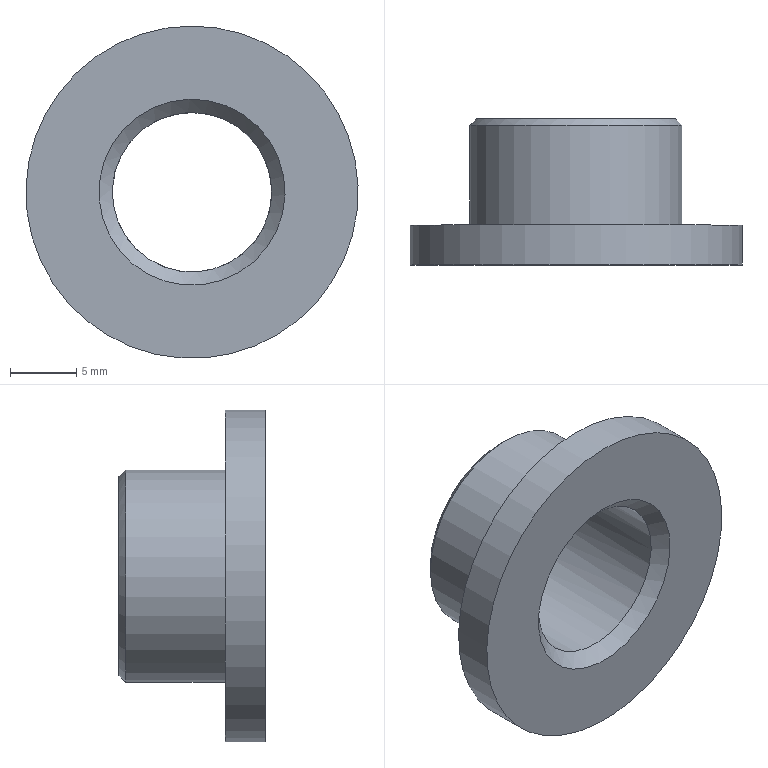Component | NX | CLHKJG_14_SHAFT_SLEEVE | 1 solid | 8 faces | box 25 x 11 x 25 mm | volume 1811 mm3 | plane 3 | cylinder 3 | cone 2 | commonest cylinder face diameters 25 x1 16 x1 12 x1
STEP:
#1=CARTESIAN_POINT('',(0.,0.,0.));
#2=DIRECTION('',(0.,0.,1.));
#3=DIRECTION('',(1.,0.,0.));
#4=AXIS2_PLACEMENT_3D('',#1,#2,#3);
#5=CARTESIAN_POINT('',(-367.568,64.665,-91.876));
#6=VERTEX_POINT('',#5);
#7=CARTESIAN_POINT('',(-360.87,64.665,-87.5));
#8=DIRECTION('',(0.,1.,0.));
#9=DIRECTION('',(-0.8372,0.,-0.5469));
#10=AXIS2_PLACEMENT_3D('',#7,#8,#9);
#11=CIRCLE('',#10,8.);
#12=CARTESIAN_POINT('',(-360.87,64.665,-87.5));
#13=DIRECTION('',(0.,1.,0.));
#14=DIRECTION('',(-0.8372,0.,-0.5469));
#15=AXIS2_PLACEMENT_3D('',#12,#13,#14);
#16=PLANE('',#15);
#17=CARTESIAN_POINT('',(0.,0.));
#18=DIRECTION('',(1.,0.));
#19=AXIS2_PLACEMENT_2D('',#17,#18);
#20=CIRCLE('',#19,8.);
#21=(GEOMETRIC_REPRESENTATION_CONTEXT(2)PARAMETRIC_REPRESENTATION_CONTEXT()REPRESENTATION_CONTEXT('',''));
#22=DEFINITIONAL_REPRESENTATION('',(#20),#21);
#23=PCURVE('',#16,#22);
#24=CARTESIAN_POINT('',(-360.87,64.665,-87.5));
#25=DIRECTION('',(0.,1.,0.));
#26=DIRECTION('',(-0.8372,0.,-0.5469));
#27=AXIS2_PLACEMENT_3D('',#24,#25,#26);
#28=CYLINDRICAL_SURFACE('',#27,8.);
#29=CARTESIAN_POINT('',(0.,0.));
#30=DIRECTION('',(1.,0.));
#31=VECTOR('',#30,1.);
#32=LINE('',#29,#31);
#33=(GEOMETRIC_REPRESENTATION_CONTEXT(2)PARAMETRIC_REPRESENTATION_CONTEXT()REPRESENTATION_CONTEXT('',''));
#34=DEFINITIONAL_REPRESENTATION('',(#32),#33);
#35=PCURVE('',#28,#34);
#36=SURFACE_CURVE('',#11,(#23,#35),.PCURVE_S1.);
#37=EDGE_CURVE('',#6,#6,#36,.T.);
#38=ORIENTED_EDGE('',*,*,#37,.F.);
#39=EDGE_LOOP('',(#38));
#40=FACE_BOUND('',#39,.T.);
#41=CARTESIAN_POINT('',(-371.335,64.665,-94.337));
#42=VERTEX_POINT('',#41);
#43=CARTESIAN_POINT('',(-360.87,64.665,-87.5));
#44=DIRECTION('',(0.,-1.,0.));
#45=DIRECTION('',(-0.8372,0.,-0.5469));
#46=AXIS2_PLACEMENT_3D('',#43,#44,#45);
#47=CIRCLE('',#46,12.5);
#48=CARTESIAN_POINT('',(12.5,-0.));
#49=CARTESIAN_POINT('',(12.5,-21.651));
#50=CARTESIAN_POINT('',(-6.25,-10.825));
#51=CARTESIAN_POINT('',(-25.,0.));
#52=CARTESIAN_POINT('',(-6.25,10.825));
#53=CARTESIAN_POINT('',(12.5,21.651));
#54=CARTESIAN_POINT('',(12.5,-0.));
#55=(BOUNDED_CURVE()B_SPLINE_CURVE(2,(#48,#49,#50,#51,#52,#53,#54),.UNSPECIFIED.,.T.,.F.)B_SPLINE_CURVE_WITH_KNOTS((1,2,2,2,2,1),(-2.094,0.,2.094,4.189,6.283,8.378),.UNSPECIFIED.)CURVE()GEOMETRIC_REPRESENTATION_ITEM()RATIONAL_B_SPLINE_CURVE((1.,0.5,1.,0.5,1.,0.5,1.))REPRESENTATION_ITEM(''));
#56=(GEOMETRIC_REPRESENTATION_CONTEXT(2)PARAMETRIC_REPRESENTATION_CONTEXT()REPRESENTATION_CONTEXT('',''));
#57=DEFINITIONAL_REPRESENTATION('',(#55),#56);
#58=PCURVE('',#16,#57);
#59=CARTESIAN_POINT('',(-360.87,61.665,-87.5));
#60=DIRECTION('',(0.,1.,0.));
#61=DIRECTION('',(-0.8372,0.,-0.5469));
#62=AXIS2_PLACEMENT_3D('',#59,#60,#61);
#63=CYLINDRICAL_SURFACE('',#62,12.5);
#64=CARTESIAN_POINT('',(6.283,3.));
#65=DIRECTION('',(-1.,0.));
#66=VECTOR('',#65,1.);
#67=LINE('',#64,#66);
#68=(GEOMETRIC_REPRESENTATION_CONTEXT(2)PARAMETRIC_REPRESENTATION_CONTEXT()REPRESENTATION_CONTEXT('',''));
#69=DEFINITIONAL_REPRESENTATION('',(#67),#68);
#70=PCURVE('',#63,#69);
#71=SURFACE_CURVE('',#47,(#58,#70),.PCURVE_S1.);
#72=EDGE_CURVE('',#42,#42,#71,.T.);
#73=ORIENTED_EDGE('',*,*,#72,.F.);
#74=EDGE_LOOP('',(#73));
#75=FACE_BOUND('',#74,.T.);
#76=ADVANCED_FACE('',(#40,#75),#16,.T.);
#77=CARTESIAN_POINT('',(-355.01,61.665,-83.671));
#78=VERTEX_POINT('',#77);
#79=CARTESIAN_POINT('',(-360.87,61.665,-87.5));
#80=DIRECTION('',(0.,1.,0.));
#81=DIRECTION('',(0.8372,0.,0.5469));
#82=AXIS2_PLACEMENT_3D('',#79,#80,#81);
#83=CIRCLE('',#82,7.);
#84=CARTESIAN_POINT('',(-360.87,61.665,-87.5));
#85=DIRECTION('',(0.,-1.,0.));
#86=DIRECTION('',(0.8372,0.,0.5469));
#87=AXIS2_PLACEMENT_3D('',#84,#85,#86);
#88=PLANE('',#87);
#89=CARTESIAN_POINT('',(7.,0.));
#90=CARTESIAN_POINT('',(7.,-12.124));
#91=CARTESIAN_POINT('',(-3.5,-6.062));
#92=CARTESIAN_POINT('',(-14.,-0.));
#93=CARTESIAN_POINT('',(-3.5,6.062));
#94=CARTESIAN_POINT('',(7.,12.124));
#95=CARTESIAN_POINT('',(7.,0.));
#96=(BOUNDED_CURVE()B_SPLINE_CURVE(2,(#89,#90,#91,#92,#93,#94,#95),.UNSPECIFIED.,.T.,.F.)B_SPLINE_CURVE_WITH_KNOTS((1,2,2,2,2,1),(-2.094,0.,2.094,4.189,6.283,8.378),.UNSPECIFIED.)CURVE()GEOMETRIC_REPRESENTATION_ITEM()RATIONAL_B_SPLINE_CURVE((1.,0.5,1.,0.5,1.,0.5,1.))REPRESENTATION_ITEM(''));
#97=(GEOMETRIC_REPRESENTATION_CONTEXT(2)PARAMETRIC_REPRESENTATION_CONTEXT()REPRESENTATION_CONTEXT('',''));
#98=DEFINITIONAL_REPRESENTATION('',(#96),#97);
#99=PCURVE('',#88,#98);
#100=CARTESIAN_POINT('',(-360.87,62.665,-87.5));
#101=DIRECTION('',(0.,-1.,0.));
#102=DIRECTION('',(0.8372,0.,0.5469));
#103=AXIS2_PLACEMENT_3D('',#100,#101,#102);
#104=CONICAL_SURFACE('',#103,6.,0.7854);
#105=CARTESIAN_POINT('',(6.283,1.));
#106=DIRECTION('',(-1.,0.));
#107=VECTOR('',#106,1.);
#108=LINE('',#105,#107);
#109=(GEOMETRIC_REPRESENTATION_CONTEXT(2)PARAMETRIC_REPRESENTATION_CONTEXT()REPRESENTATION_CONTEXT('',''));
#110=DEFINITIONAL_REPRESENTATION('',(#108),#109);
#111=PCURVE('',#104,#110);
#112=SURFACE_CURVE('',#83,(#99,#111),.PCURVE_S1.);
#113=EDGE_CURVE('',#78,#78,#112,.T.);
#114=ORIENTED_EDGE('',*,*,#113,.T.);
#115=EDGE_LOOP('',(#114));
#116=FACE_BOUND('',#115,.T.);
#117=CARTESIAN_POINT('',(-371.335,61.665,-94.337));
#118=VERTEX_POINT('',#117);
#119=CARTESIAN_POINT('',(-360.87,61.665,-87.5));
#120=DIRECTION('',(0.,1.,0.));
#121=DIRECTION('',(-0.8372,0.,-0.5469));
#122=AXIS2_PLACEMENT_3D('',#119,#120,#121);
#123=CIRCLE('',#122,12.5);
#124=CARTESIAN_POINT('',(-12.5,-0.));
#125=CARTESIAN_POINT('',(-12.5,21.651));
#126=CARTESIAN_POINT('',(6.25,10.825));
#127=CARTESIAN_POINT('',(25.,0.));
#128=CARTESIAN_POINT('',(6.25,-10.825));
#129=CARTESIAN_POINT('',(-12.5,-21.651));
#130=CARTESIAN_POINT('',(-12.5,-0.));
#131=(BOUNDED_CURVE()B_SPLINE_CURVE(2,(#124,#125,#126,#127,#128,#129,#130),.UNSPECIFIED.,.T.,.F.)B_SPLINE_CURVE_WITH_KNOTS((1,2,2,2,2,1),(-2.094,0.,2.094,4.189,6.283,8.378),.UNSPECIFIED.)CURVE()GEOMETRIC_REPRESENTATION_ITEM()RATIONAL_B_SPLINE_CURVE((1.,0.5,1.,0.5,1.,0.5,1.))REPRESENTATION_ITEM(''));
#132=(GEOMETRIC_REPRESENTATION_CONTEXT(2)PARAMETRIC_REPRESENTATION_CONTEXT()REPRESENTATION_CONTEXT('',''));
#133=DEFINITIONAL_REPRESENTATION('',(#131),#132);
#134=PCURVE('',#88,#133);
#135=CARTESIAN_POINT('',(0.,0.));
#136=DIRECTION('',(1.,0.));
#137=VECTOR('',#136,1.);
#138=LINE('',#135,#137);
#139=(GEOMETRIC_REPRESENTATION_CONTEXT(2)PARAMETRIC_REPRESENTATION_CONTEXT()REPRESENTATION_CONTEXT('',''));
#140=DEFINITIONAL_REPRESENTATION('',(#138),#139);
#141=PCURVE('',#63,#140);
#142=SURFACE_CURVE('',#123,(#134,#141),.PCURVE_S1.);
#143=EDGE_CURVE('',#118,#118,#142,.T.);
#144=ORIENTED_EDGE('',*,*,#143,.F.);
#145=EDGE_LOOP('',(#144));
#146=FACE_BOUND('',#145,.T.);
#147=ADVANCED_FACE('',(#116,#146),#88,.T.);
#148=ORIENTED_EDGE('',*,*,#72,.T.);
#149=CARTESIAN_POINT('',(-371.335,61.665,-94.337));
#150=CARTESIAN_POINT('',(-371.335,64.665,-94.337));
#151=B_SPLINE_CURVE_WITH_KNOTS('',1,(#149,#150),.UNSPECIFIED.,.F.,.F.,(2,2),(0.,3.),.PIECEWISE_BEZIER_KNOTS.);
#152=CARTESIAN_POINT('',(0.,0.));
#153=DIRECTION('',(0.,1.));
#154=VECTOR('',#153,1.);
#155=LINE('',#152,#154);
#156=(GEOMETRIC_REPRESENTATION_CONTEXT(2)PARAMETRIC_REPRESENTATION_CONTEXT()REPRESENTATION_CONTEXT('',''));
#157=DEFINITIONAL_REPRESENTATION('',(#155),#156);
#158=PCURVE('',#63,#157);
#159=CARTESIAN_POINT('',(6.283,0.));
#160=DIRECTION('',(0.,1.));
#161=VECTOR('',#160,1.);
#162=LINE('',#159,#161);
#163=(GEOMETRIC_REPRESENTATION_CONTEXT(2)PARAMETRIC_REPRESENTATION_CONTEXT()REPRESENTATION_CONTEXT('',''));
#164=DEFINITIONAL_REPRESENTATION('',(#162),#163);
#165=PCURVE('',#63,#164);
#166=SEAM_CURVE('',#151,(#158,#165),.PCURVE_S1.);
#167=EDGE_CURVE('',#118,#42,#166,.T.);
#168=ORIENTED_EDGE('',*,*,#167,.F.);
#169=ORIENTED_EDGE('',*,*,#143,.T.);
#170=ORIENTED_EDGE('',*,*,#167,.T.);
#171=EDGE_LOOP('',(#148,#168,#169,#170));
#172=FACE_BOUND('',#171,.T.);
#173=ADVANCED_FACE('',(#172),#63,.T.);
#174=CARTESIAN_POINT('',(-365.893,72.665,-90.782));
#175=VERTEX_POINT('',#174);
#176=CARTESIAN_POINT('',(-360.87,72.665,-87.5));
#177=DIRECTION('',(0.,-1.,0.));
#178=DIRECTION('',(-0.8372,0.,-0.5469));
#179=AXIS2_PLACEMENT_3D('',#176,#177,#178);
#180=CIRCLE('',#179,6.);
#181=CARTESIAN_POINT('',(-360.87,72.665,-87.5));
#182=DIRECTION('',(0.,1.,0.));
#183=DIRECTION('',(-0.8372,0.,-0.5469));
#184=AXIS2_PLACEMENT_3D('',#181,#182,#183);
#185=PLANE('',#184);
#186=CARTESIAN_POINT('',(6.,-0.));
#187=CARTESIAN_POINT('',(6.,-10.392));
#188=CARTESIAN_POINT('',(-3.,-5.196));
#189=CARTESIAN_POINT('',(-12.,0.));
#190=CARTESIAN_POINT('',(-3.,5.196));
#191=CARTESIAN_POINT('',(6.,10.392));
#192=CARTESIAN_POINT('',(6.,-0.));
#193=(BOUNDED_CURVE()B_SPLINE_CURVE(2,(#186,#187,#188,#189,#190,#191,#192),.UNSPECIFIED.,.T.,.F.)B_SPLINE_CURVE_WITH_KNOTS((1,2,2,2,2,1),(-2.094,0.,2.094,4.189,6.283,8.378),.UNSPECIFIED.)CURVE()GEOMETRIC_REPRESENTATION_ITEM()RATIONAL_B_SPLINE_CURVE((1.,0.5,1.,0.5,1.,0.5,1.))REPRESENTATION_ITEM(''));
#194=(GEOMETRIC_REPRESENTATION_CONTEXT(2)PARAMETRIC_REPRESENTATION_CONTEXT()REPRESENTATION_CONTEXT('',''));
#195=DEFINITIONAL_REPRESENTATION('',(#193),#194);
#196=PCURVE('',#185,#195);
#197=CARTESIAN_POINT('',(-360.87,72.665,-87.5));
#198=DIRECTION('',(0.,-1.,0.));
#199=DIRECTION('',(-0.8372,0.,-0.5469));
#200=AXIS2_PLACEMENT_3D('',#197,#198,#199);
#201=CYLINDRICAL_SURFACE('',#200,6.);
#202=CARTESIAN_POINT('',(0.,0.));
#203=DIRECTION('',(1.,0.));
#204=VECTOR('',#203,1.);
#205=LINE('',#202,#204);
#206=(GEOMETRIC_REPRESENTATION_CONTEXT(2)PARAMETRIC_REPRESENTATION_CONTEXT()REPRESENTATION_CONTEXT('',''));
#207=DEFINITIONAL_REPRESENTATION('',(#205),#206);
#208=PCURVE('',#201,#207);
#209=SURFACE_CURVE('',#180,(#196,#208),.PCURVE_S1.);
#210=EDGE_CURVE('',#175,#175,#209,.T.);
#211=ORIENTED_EDGE('',*,*,#210,.T.);
#212=EDGE_LOOP('',(#211));
#213=FACE_BOUND('',#212,.T.);
#214=CARTESIAN_POINT('',(-367.149,72.665,-91.602));
#215=VERTEX_POINT('',#214);
#216=CARTESIAN_POINT('',(-360.87,72.665,-87.5));
#217=DIRECTION('',(0.,1.,0.));
#218=DIRECTION('',(-0.8372,0.,-0.5469));
#219=AXIS2_PLACEMENT_3D('',#216,#217,#218);
#220=CIRCLE('',#219,7.5);
#221=CARTESIAN_POINT('',(0.,0.));
#222=DIRECTION('',(1.,0.));
#223=AXIS2_PLACEMENT_2D('',#221,#222);
#224=CIRCLE('',#223,7.5);
#225=(GEOMETRIC_REPRESENTATION_CONTEXT(2)PARAMETRIC_REPRESENTATION_CONTEXT()REPRESENTATION_CONTEXT('',''));
#226=DEFINITIONAL_REPRESENTATION('',(#224),#225);
#227=PCURVE('',#185,#226);
#228=CARTESIAN_POINT('',(-360.87,72.165,-87.5));
#229=DIRECTION('',(0.,-1.,0.));
#230=DIRECTION('',(0.8372,0.,0.5469));
#231=AXIS2_PLACEMENT_3D('',#228,#229,#230);
#232=CONICAL_SURFACE('',#231,8.,0.7854);
#233=CARTESIAN_POINT('',(9.425,-0.5));
#234=DIRECTION('',(-1.,0.));
#235=VECTOR('',#234,1.);
#236=LINE('',#233,#235);
#237=(GEOMETRIC_REPRESENTATION_CONTEXT(2)PARAMETRIC_REPRESENTATION_CONTEXT()REPRESENTATION_CONTEXT('',''));
#238=DEFINITIONAL_REPRESENTATION('',(#236),#237);
#239=PCURVE('',#232,#238);
#240=SURFACE_CURVE('',#220,(#227,#239),.PCURVE_S1.);
#241=EDGE_CURVE('',#215,#215,#240,.T.);
#242=ORIENTED_EDGE('',*,*,#241,.T.);
#243=EDGE_LOOP('',(#242));
#244=FACE_BOUND('',#243,.T.);
#245=ADVANCED_FACE('',(#213,#244),#185,.T.);
#246=CARTESIAN_POINT('',(-367.568,72.165,-91.876));
#247=VERTEX_POINT('',#246);
#248=CARTESIAN_POINT('',(-360.87,72.165,-87.5));
#249=DIRECTION('',(0.,-1.,0.));
#250=DIRECTION('',(-0.8372,0.,-0.5469));
#251=AXIS2_PLACEMENT_3D('',#248,#249,#250);
#252=CIRCLE('',#251,8.);
#253=CARTESIAN_POINT('',(6.283,7.5));
#254=DIRECTION('',(-1.,0.));
#255=VECTOR('',#254,1.);
#256=LINE('',#253,#255);
#257=(GEOMETRIC_REPRESENTATION_CONTEXT(2)PARAMETRIC_REPRESENTATION_CONTEXT()REPRESENTATION_CONTEXT('',''));
#258=DEFINITIONAL_REPRESENTATION('',(#256),#257);
#259=PCURVE('',#28,#258);
#260=CARTESIAN_POINT('',(3.142,0.));
#261=DIRECTION('',(1.,0.));
#262=VECTOR('',#261,1.);
#263=LINE('',#260,#262);
#264=(GEOMETRIC_REPRESENTATION_CONTEXT(2)PARAMETRIC_REPRESENTATION_CONTEXT()REPRESENTATION_CONTEXT('',''));
#265=DEFINITIONAL_REPRESENTATION('',(#263),#264);
#266=PCURVE('',#232,#265);
#267=SURFACE_CURVE('',#252,(#259,#266),.PCURVE_S1.);
#268=EDGE_CURVE('',#247,#247,#267,.T.);
#269=ORIENTED_EDGE('',*,*,#268,.T.);
#270=CARTESIAN_POINT('',(-367.568,64.665,-91.876));
#271=CARTESIAN_POINT('',(-367.568,72.165,-91.876));
#272=B_SPLINE_CURVE_WITH_KNOTS('',1,(#270,#271),.UNSPECIFIED.,.F.,.F.,(2,2),(0.,7.5),.PIECEWISE_BEZIER_KNOTS.);
#273=CARTESIAN_POINT('',(0.,0.));
#274=DIRECTION('',(0.,1.));
#275=VECTOR('',#274,1.);
#276=LINE('',#273,#275);
#277=(GEOMETRIC_REPRESENTATION_CONTEXT(2)PARAMETRIC_REPRESENTATION_CONTEXT()REPRESENTATION_CONTEXT('',''));
#278=DEFINITIONAL_REPRESENTATION('',(#276),#277);
#279=PCURVE('',#28,#278);
#280=CARTESIAN_POINT('',(6.283,0.));
#281=DIRECTION('',(0.,1.));
#282=VECTOR('',#281,1.);
#283=LINE('',#280,#282);
#284=(GEOMETRIC_REPRESENTATION_CONTEXT(2)PARAMETRIC_REPRESENTATION_CONTEXT()REPRESENTATION_CONTEXT('',''));
#285=DEFINITIONAL_REPRESENTATION('',(#283),#284);
#286=PCURVE('',#28,#285);
#287=SEAM_CURVE('',#272,(#279,#286),.PCURVE_S1.);
#288=EDGE_CURVE('',#6,#247,#287,.T.);
#289=ORIENTED_EDGE('',*,*,#288,.F.);
#290=ORIENTED_EDGE('',*,*,#37,.T.);
#291=ORIENTED_EDGE('',*,*,#288,.T.);
#292=EDGE_LOOP('',(#269,#289,#290,#291));
#293=FACE_BOUND('',#292,.T.);
#294=ADVANCED_FACE('',(#293),#28,.T.);
#295=ORIENTED_EDGE('',*,*,#241,.F.);
#296=CARTESIAN_POINT('',(-367.149,72.665,-91.602));
#297=CARTESIAN_POINT('',(-367.568,72.165,-91.876));
#298=B_SPLINE_CURVE_WITH_KNOTS('',1,(#296,#297),.UNSPECIFIED.,.F.,.F.,(2,2),(-0.7071,0.),.PIECEWISE_BEZIER_KNOTS.);
#299=CARTESIAN_POINT('',(9.425,0.));
#300=DIRECTION('',(0.,1.));
#301=VECTOR('',#300,1.);
#302=LINE('',#299,#301);
#303=(GEOMETRIC_REPRESENTATION_CONTEXT(2)PARAMETRIC_REPRESENTATION_CONTEXT()REPRESENTATION_CONTEXT('',''));
#304=DEFINITIONAL_REPRESENTATION('',(#302),#303);
#305=PCURVE('',#232,#304);
#306=CARTESIAN_POINT('',(3.142,0.));
#307=DIRECTION('',(0.,1.));
#308=VECTOR('',#307,1.);
#309=LINE('',#306,#308);
#310=(GEOMETRIC_REPRESENTATION_CONTEXT(2)PARAMETRIC_REPRESENTATION_CONTEXT()REPRESENTATION_CONTEXT('',''));
#311=DEFINITIONAL_REPRESENTATION('',(#309),#310);
#312=PCURVE('',#232,#311);
#313=SEAM_CURVE('',#298,(#305,#312),.PCURVE_S1.);
#314=EDGE_CURVE('',#215,#247,#313,.T.);
#315=ORIENTED_EDGE('',*,*,#314,.T.);
#316=ORIENTED_EDGE('',*,*,#268,.F.);
#317=ORIENTED_EDGE('',*,*,#314,.F.);
#318=EDGE_LOOP('',(#295,#315,#316,#317));
#319=FACE_BOUND('',#318,.T.);
#320=ADVANCED_FACE('',(#319),#232,.T.);
#321=CARTESIAN_POINT('',(-365.893,62.665,-90.782));
#322=VERTEX_POINT('',#321);
#323=CARTESIAN_POINT('',(-355.847,62.665,-84.218));
#324=VERTEX_POINT('',#323);
#325=CARTESIAN_POINT('',(-360.87,62.665,-87.5));
#326=DIRECTION('',(0.,-1.,0.));
#327=DIRECTION('',(0.8372,0.,0.5469));
#328=AXIS2_PLACEMENT_3D('',#325,#326,#327);
#329=CIRCLE('',#328,6.);
#330=CARTESIAN_POINT('',(-3.142,10.));
#331=DIRECTION('',(1.,0.));
#332=VECTOR('',#331,1.);
#333=LINE('',#330,#332);
#334=(GEOMETRIC_REPRESENTATION_CONTEXT(2)PARAMETRIC_REPRESENTATION_CONTEXT()REPRESENTATION_CONTEXT('',''));
#335=DEFINITIONAL_REPRESENTATION('',(#333),#334);
#336=PCURVE('',#201,#335);
#337=CARTESIAN_POINT('',(0.,0.));
#338=DIRECTION('',(1.,0.));
#339=VECTOR('',#338,1.);
#340=LINE('',#337,#339);
#341=(GEOMETRIC_REPRESENTATION_CONTEXT(2)PARAMETRIC_REPRESENTATION_CONTEXT()REPRESENTATION_CONTEXT('',''));
#342=DEFINITIONAL_REPRESENTATION('',(#340),#341);
#343=PCURVE('',#104,#342);
#344=SURFACE_CURVE('',#329,(#336,#343),.PCURVE_S1.);
#345=EDGE_CURVE('',#322,#324,#344,.T.);
#346=ORIENTED_EDGE('',*,*,#345,.F.);
#347=CARTESIAN_POINT('',(-365.893,72.665,-90.782));
#348=CARTESIAN_POINT('',(-365.893,62.665,-90.782));
#349=B_SPLINE_CURVE_WITH_KNOTS('',1,(#347,#348),.UNSPECIFIED.,.F.,.F.,(2,2),(0.,10.),.PIECEWISE_BEZIER_KNOTS.);
#350=CARTESIAN_POINT('',(0.,0.));
#351=DIRECTION('',(0.,1.));
#352=VECTOR('',#351,1.);
#353=LINE('',#350,#352);
#354=(GEOMETRIC_REPRESENTATION_CONTEXT(2)PARAMETRIC_REPRESENTATION_CONTEXT()REPRESENTATION_CONTEXT('',''));
#355=DEFINITIONAL_REPRESENTATION('',(#353),#354);
#356=PCURVE('',#201,#355);
#357=CARTESIAN_POINT('',(6.283,0.));
#358=DIRECTION('',(0.,1.));
#359=VECTOR('',#358,1.);
#360=LINE('',#357,#359);
#361=(GEOMETRIC_REPRESENTATION_CONTEXT(2)PARAMETRIC_REPRESENTATION_CONTEXT()REPRESENTATION_CONTEXT('',''));
#362=DEFINITIONAL_REPRESENTATION('',(#360),#361);
#363=PCURVE('',#201,#362);
#364=SEAM_CURVE('',#349,(#356,#363),.PCURVE_S1.);
#365=EDGE_CURVE('',#175,#322,#364,.T.);
#366=ORIENTED_EDGE('',*,*,#365,.F.);
#367=ORIENTED_EDGE('',*,*,#210,.T.);
#368=ORIENTED_EDGE('',*,*,#365,.T.);
#369=CARTESIAN_POINT('',(-360.87,62.665,-87.5));
#370=DIRECTION('',(0.,-1.,0.));
#371=DIRECTION('',(0.8372,0.,0.5469));
#372=AXIS2_PLACEMENT_3D('',#369,#370,#371);
#373=CIRCLE('',#372,6.);
#374=CARTESIAN_POINT('',(3.142,10.));
#375=DIRECTION('',(1.,0.));
#376=VECTOR('',#375,1.);
#377=LINE('',#374,#376);
#378=(GEOMETRIC_REPRESENTATION_CONTEXT(2)PARAMETRIC_REPRESENTATION_CONTEXT()REPRESENTATION_CONTEXT('',''));
#379=DEFINITIONAL_REPRESENTATION('',(#377),#378);
#380=PCURVE('',#201,#379);
#381=CARTESIAN_POINT('',(0.,0.));
#382=DIRECTION('',(1.,0.));
#383=VECTOR('',#382,1.);
#384=LINE('',#381,#383);
#385=(GEOMETRIC_REPRESENTATION_CONTEXT(2)PARAMETRIC_REPRESENTATION_CONTEXT()REPRESENTATION_CONTEXT('',''));
#386=DEFINITIONAL_REPRESENTATION('',(#384),#385);
#387=PCURVE('',#104,#386);
#388=SURFACE_CURVE('',#373,(#380,#387),.PCURVE_S1.);
#389=EDGE_CURVE('',#324,#322,#388,.T.);
#390=ORIENTED_EDGE('',*,*,#389,.F.);
#391=EDGE_LOOP('',(#346,#366,#367,#368,#390));
#392=FACE_BOUND('',#391,.F.);
#393=ADVANCED_FACE('',(#392),#201,.F.);
#394=ORIENTED_EDGE('',*,*,#113,.T.);
#395=CARTESIAN_POINT('',(-355.847,62.665,-84.218));
#396=CARTESIAN_POINT('',(-355.01,61.665,-83.671));
#397=B_SPLINE_CURVE_WITH_KNOTS('',1,(#395,#396),.UNSPECIFIED.,.F.,.F.,(2,2),(0.,1.414),.PIECEWISE_BEZIER_KNOTS.);
#398=CARTESIAN_POINT('',(0.,0.));
#399=DIRECTION('',(0.,1.));
#400=VECTOR('',#399,1.);
#401=LINE('',#398,#400);
#402=(GEOMETRIC_REPRESENTATION_CONTEXT(2)PARAMETRIC_REPRESENTATION_CONTEXT()REPRESENTATION_CONTEXT('',''));
#403=DEFINITIONAL_REPRESENTATION('',(#401),#402);
#404=PCURVE('',#104,#403);
#405=CARTESIAN_POINT('',(6.283,0.));
#406=DIRECTION('',(0.,1.));
#407=VECTOR('',#406,1.);
#408=LINE('',#405,#407);
#409=(GEOMETRIC_REPRESENTATION_CONTEXT(2)PARAMETRIC_REPRESENTATION_CONTEXT()REPRESENTATION_CONTEXT('',''));
#410=DEFINITIONAL_REPRESENTATION('',(#408),#409);
#411=PCURVE('',#104,#410);
#412=SEAM_CURVE('',#397,(#404,#411),.PCURVE_S1.);
#413=EDGE_CURVE('',#324,#78,#412,.T.);
#414=ORIENTED_EDGE('',*,*,#413,.F.);
#415=ORIENTED_EDGE('',*,*,#389,.T.);
#416=ORIENTED_EDGE('',*,*,#345,.T.);
#417=ORIENTED_EDGE('',*,*,#413,.T.);
#418=EDGE_LOOP('',(#394,#414,#415,#416,#417));
#419=FACE_BOUND('',#418,.F.);
#420=ADVANCED_FACE('',(#419),#104,.F.);
#421=CLOSED_SHELL('',(#76,#147,#173,#245,#294,#320,#393,#420));
#422=MANIFOLD_SOLID_BREP('',#421);
#423=(LENGTH_UNIT()NAMED_UNIT(*)SI_UNIT(.MILLI.,.METRE.));
#424=UNCERTAINTY_MEASURE_WITH_UNIT(LENGTH_MEASURE(0.00001),#423,'','');
#425=(NAMED_UNIT(*)PLANE_ANGLE_UNIT()SI_UNIT($,.RADIAN.));
#426=(NAMED_UNIT(*)SI_UNIT($,.STERADIAN.)SOLID_ANGLE_UNIT());
#427=(GEOMETRIC_REPRESENTATION_CONTEXT(3)GLOBAL_UNCERTAINTY_ASSIGNED_CONTEXT((#424))GLOBAL_UNIT_ASSIGNED_CONTEXT((#423,#425,#426))REPRESENTATION_CONTEXT('',''));
#428=ADVANCED_BREP_SHAPE_REPRESENTATION('',(#4,#422),#427);